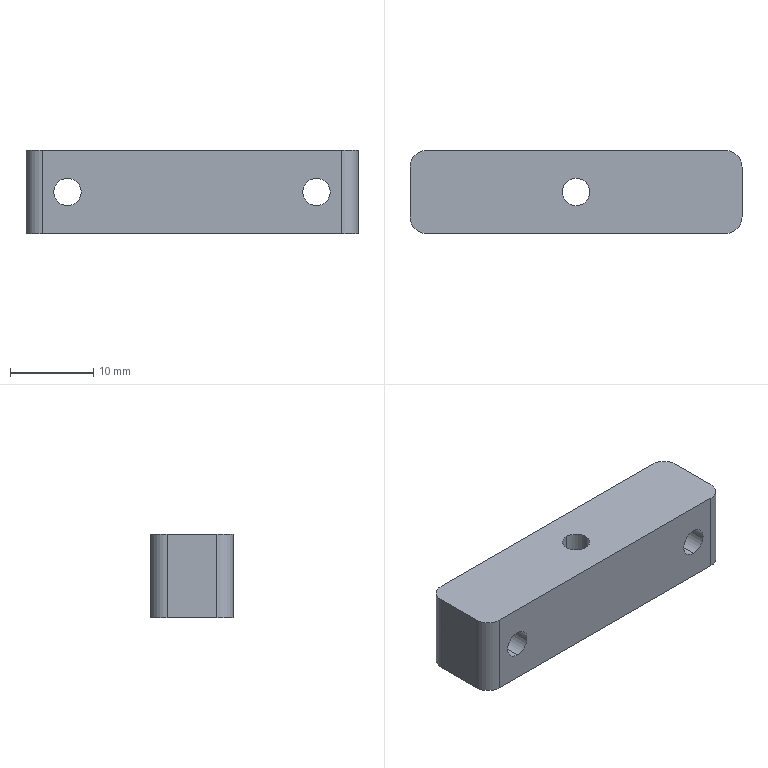CAM job | Mastercam | mm | 10 operations | part box 40 x 10 x 10
1. Facing | 23 - 50 平铣刀
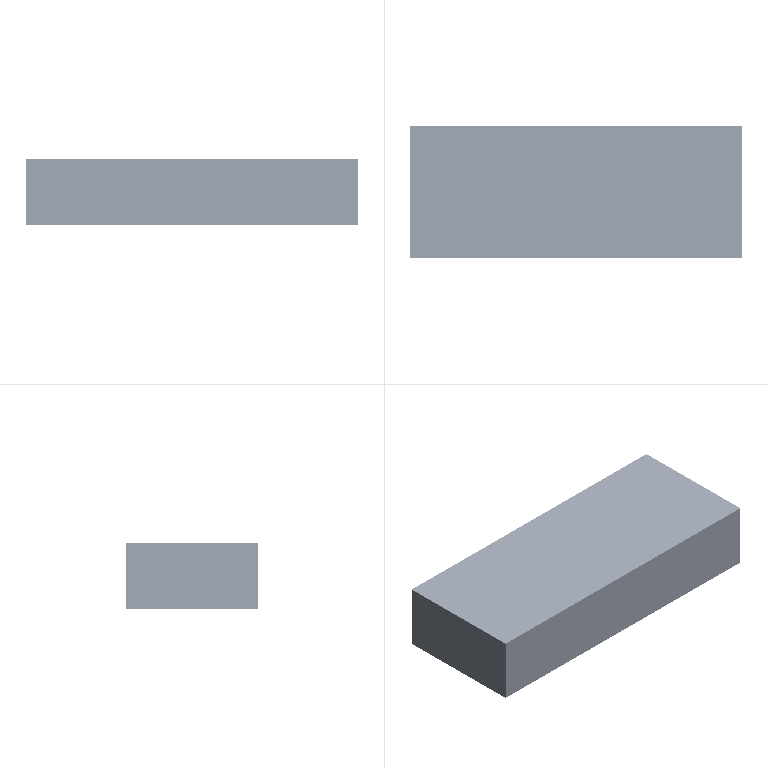2. 2D High Speed (2D Dynamic Mill) | 12 - 12 平铣刀
3. Contour (2D) | 8 - 8 平铣刀
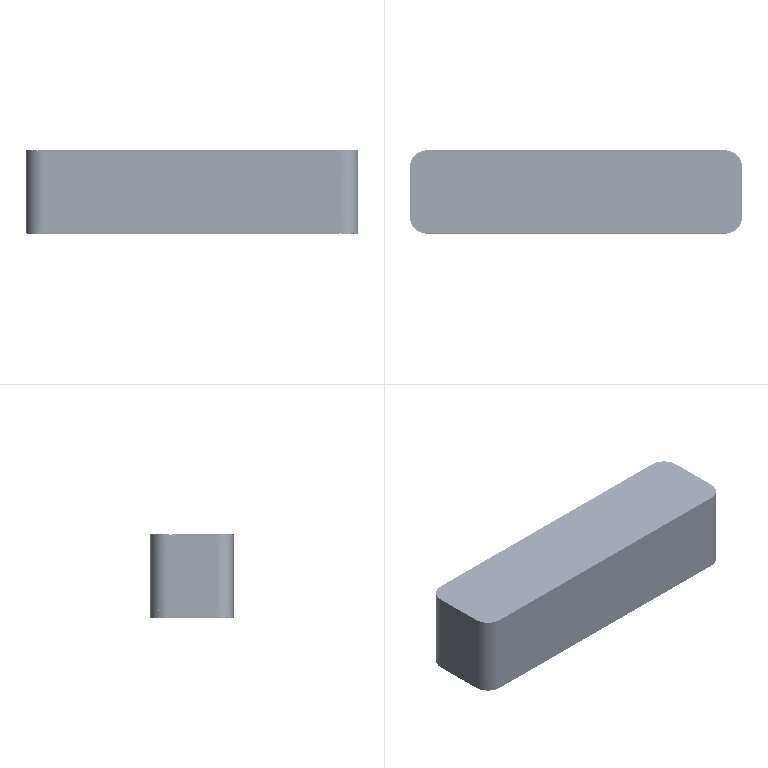4. Facing | 8 - 8 平铣刀
5. Contour (2D chamfer) | 7 - 4 倒角刀
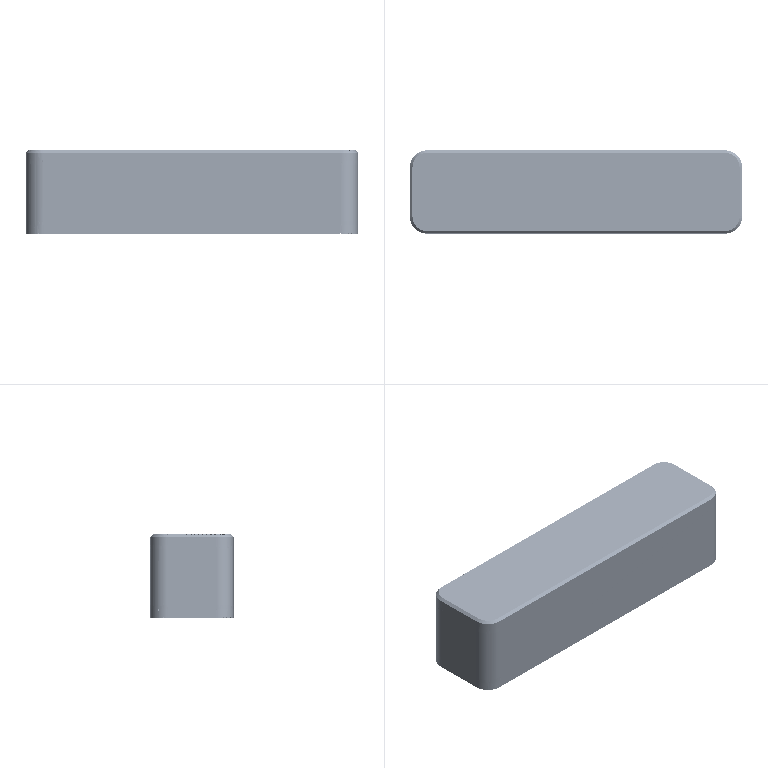6. Drill/Counterbore | 7 - 4 倒角刀
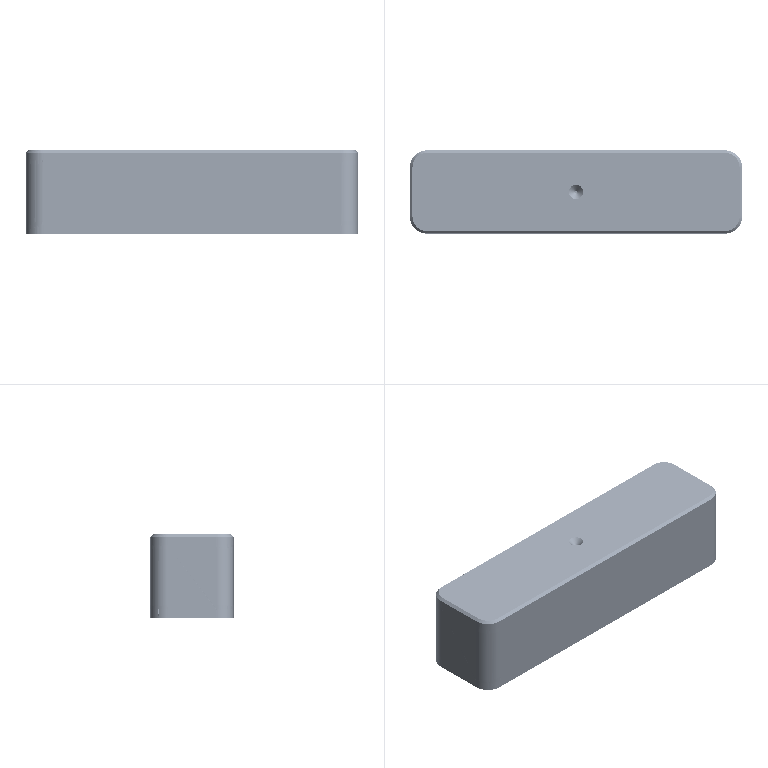7. Facing | 23 - 50 平铣刀
8. Facing | 8 - 8 平铣刀
9. Contour (2D chamfer) | 7 - 4 倒角刀
10. Drill/Counterbore | 7 - 4 倒角刀